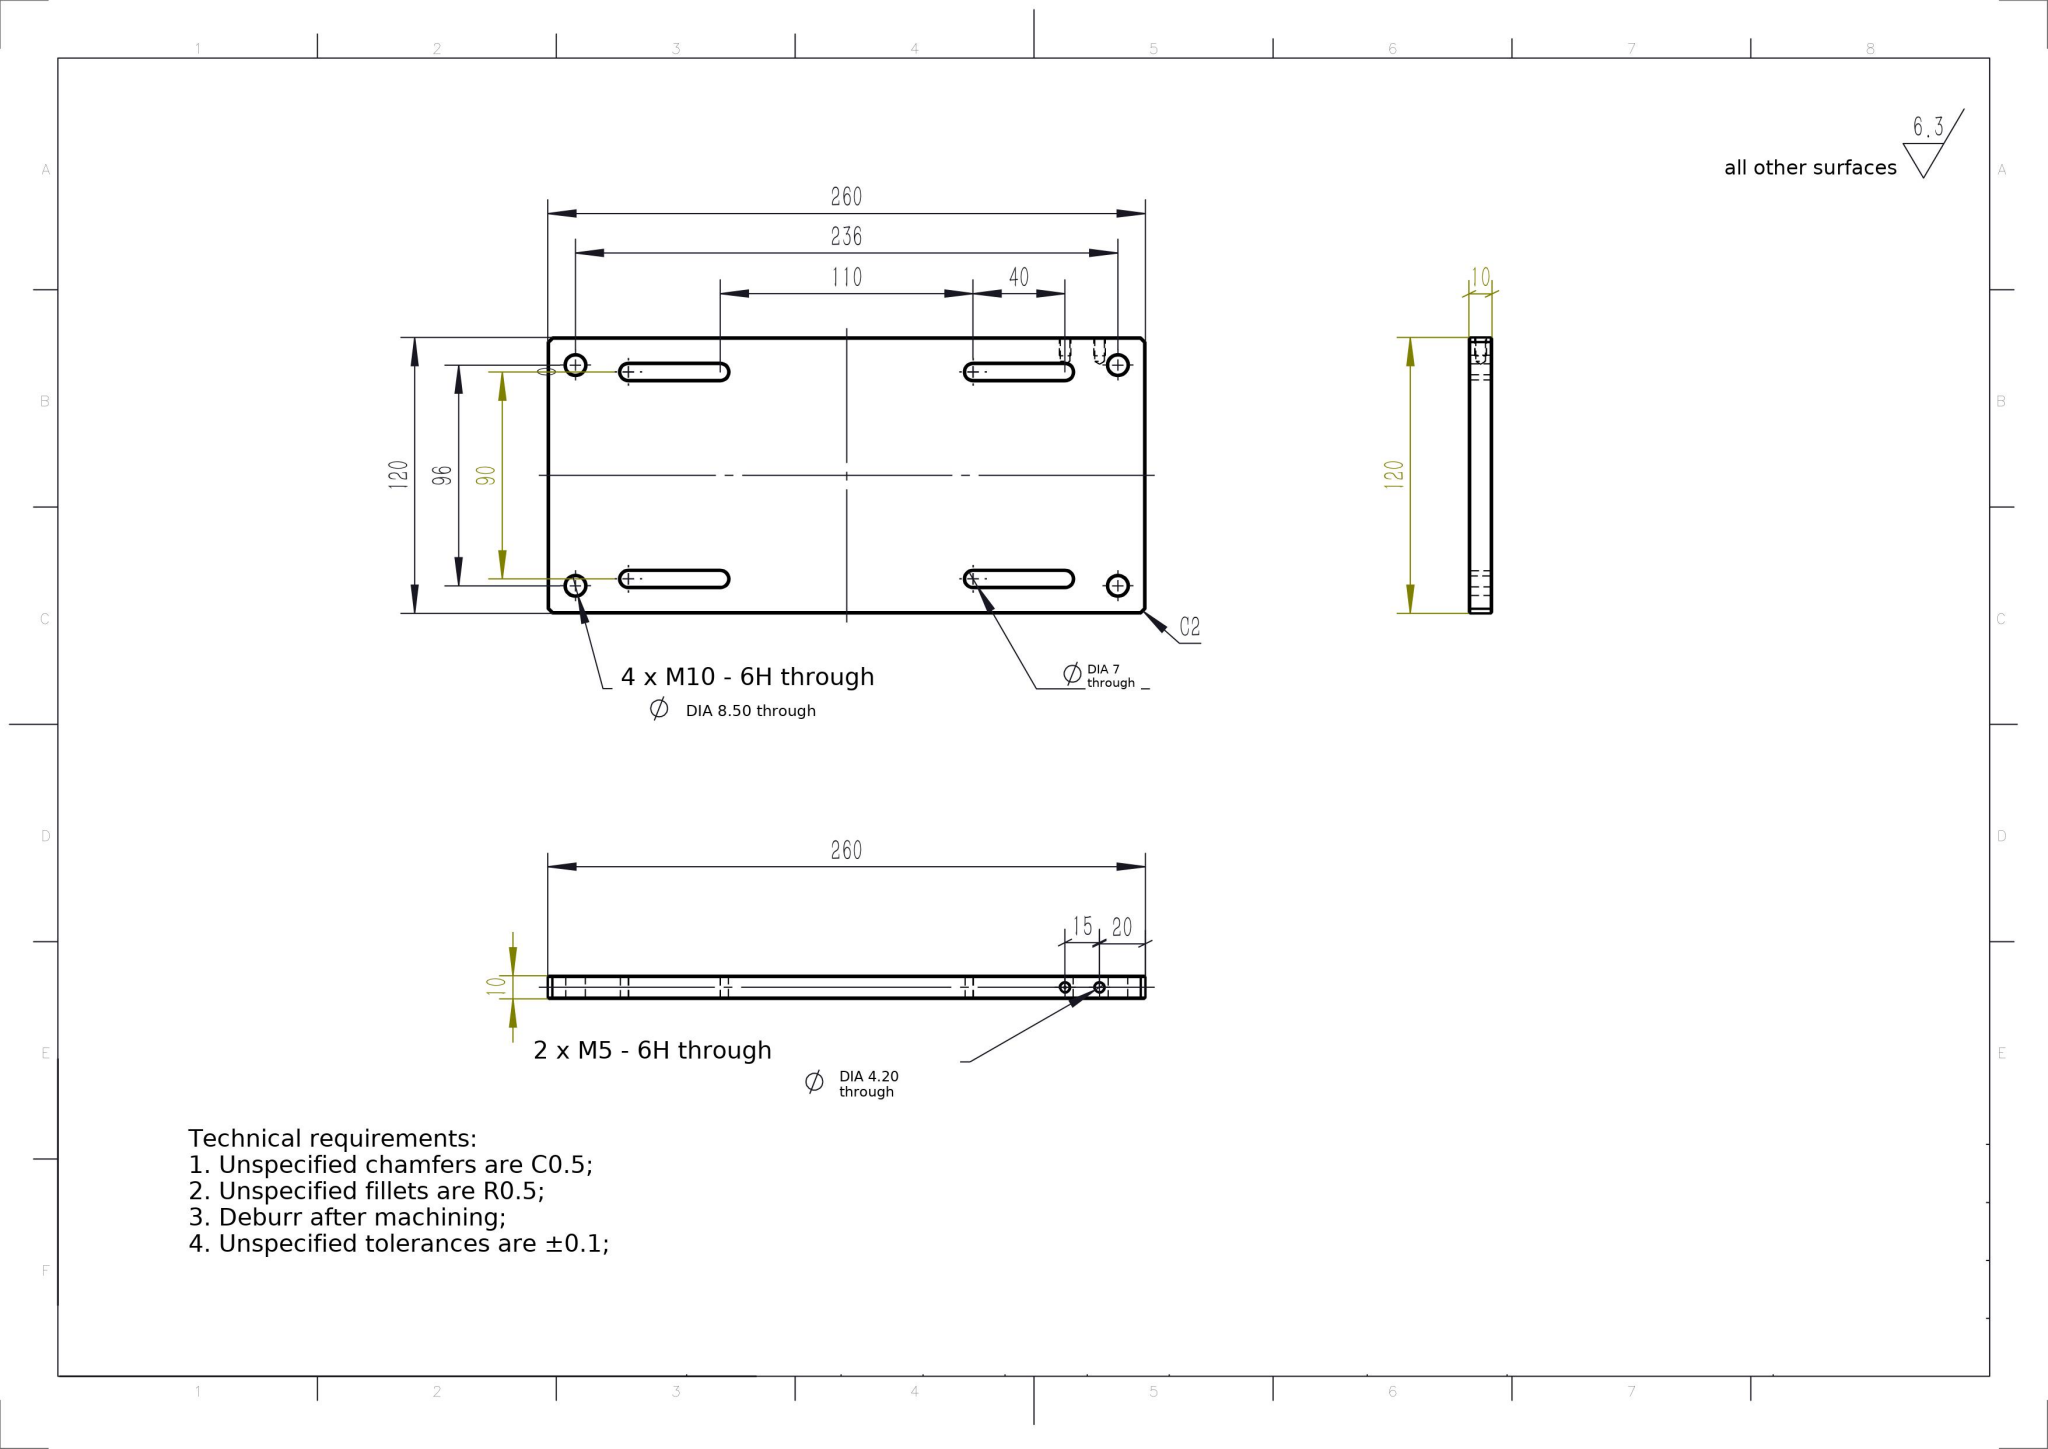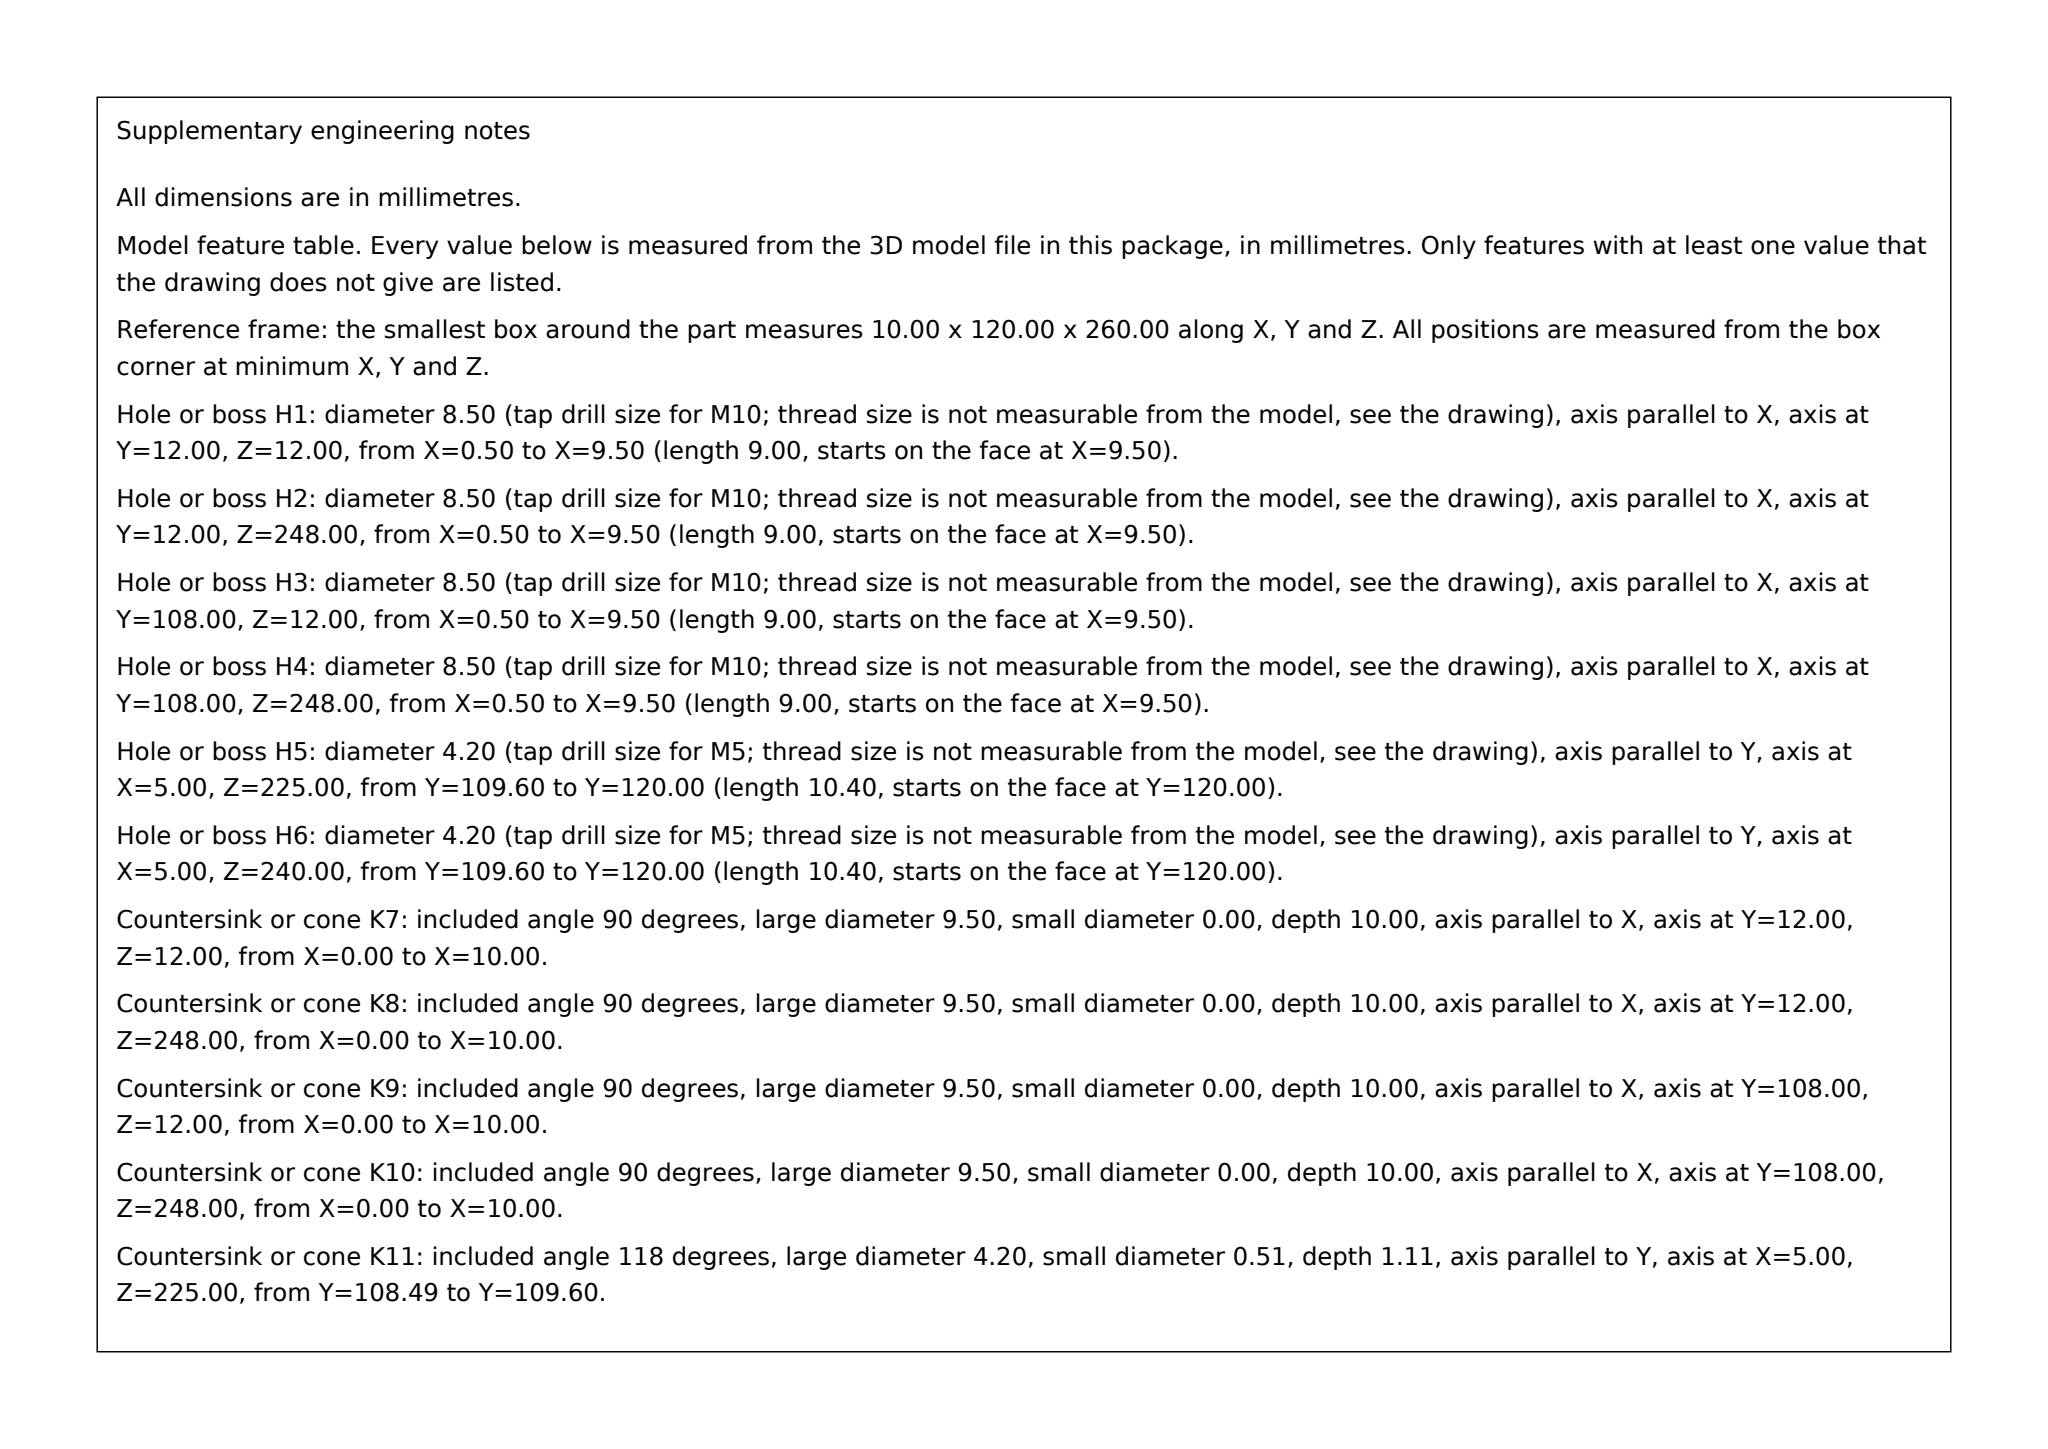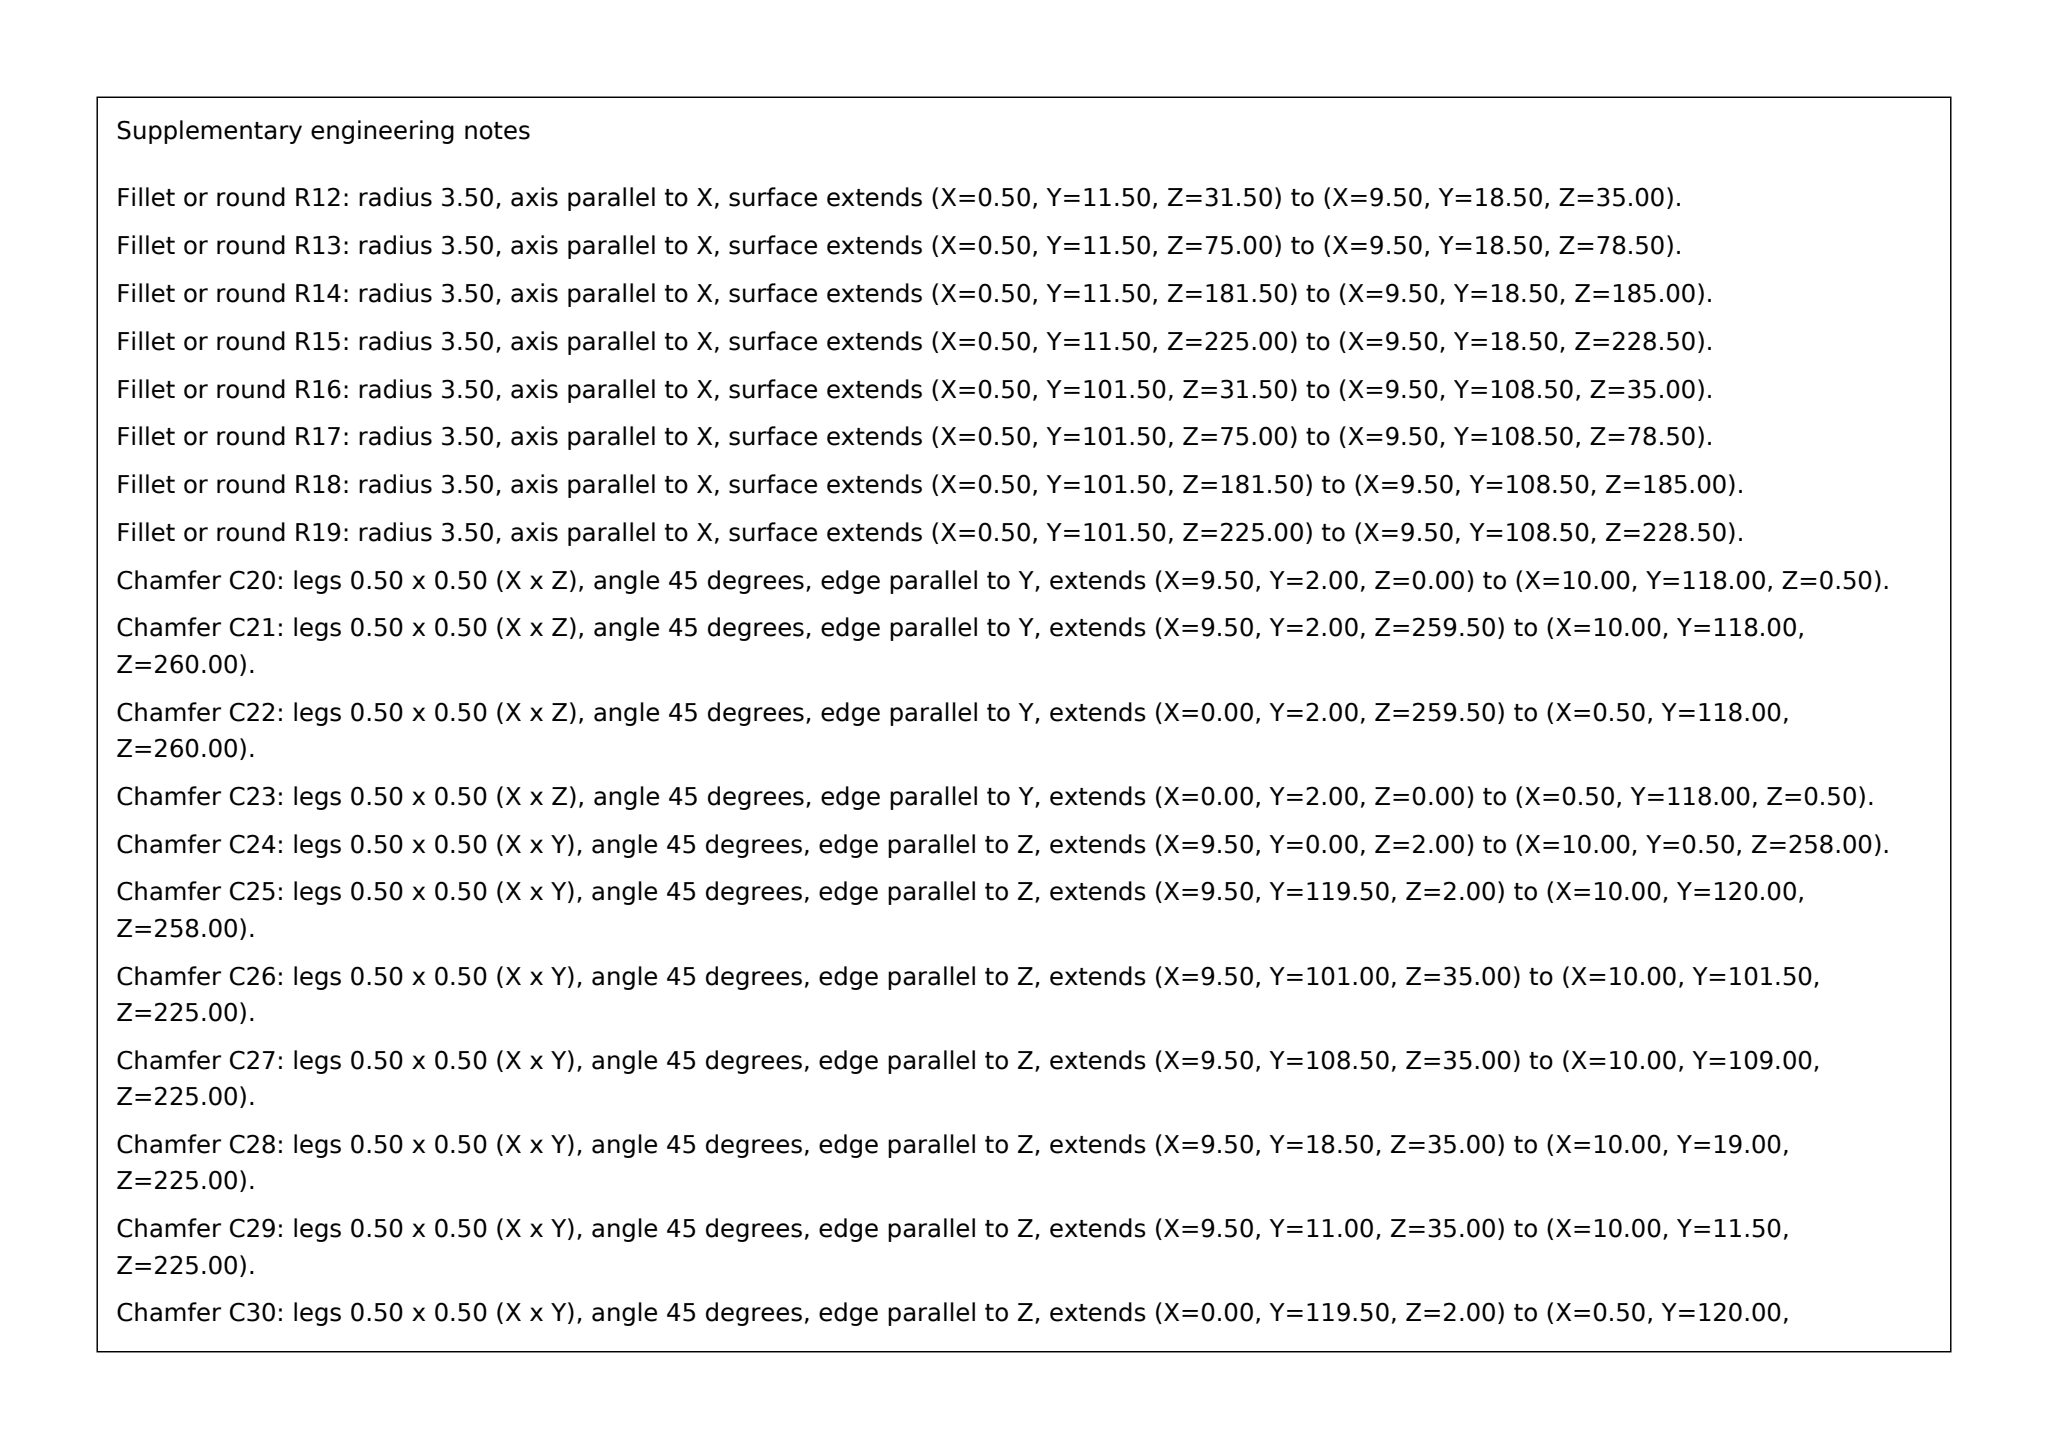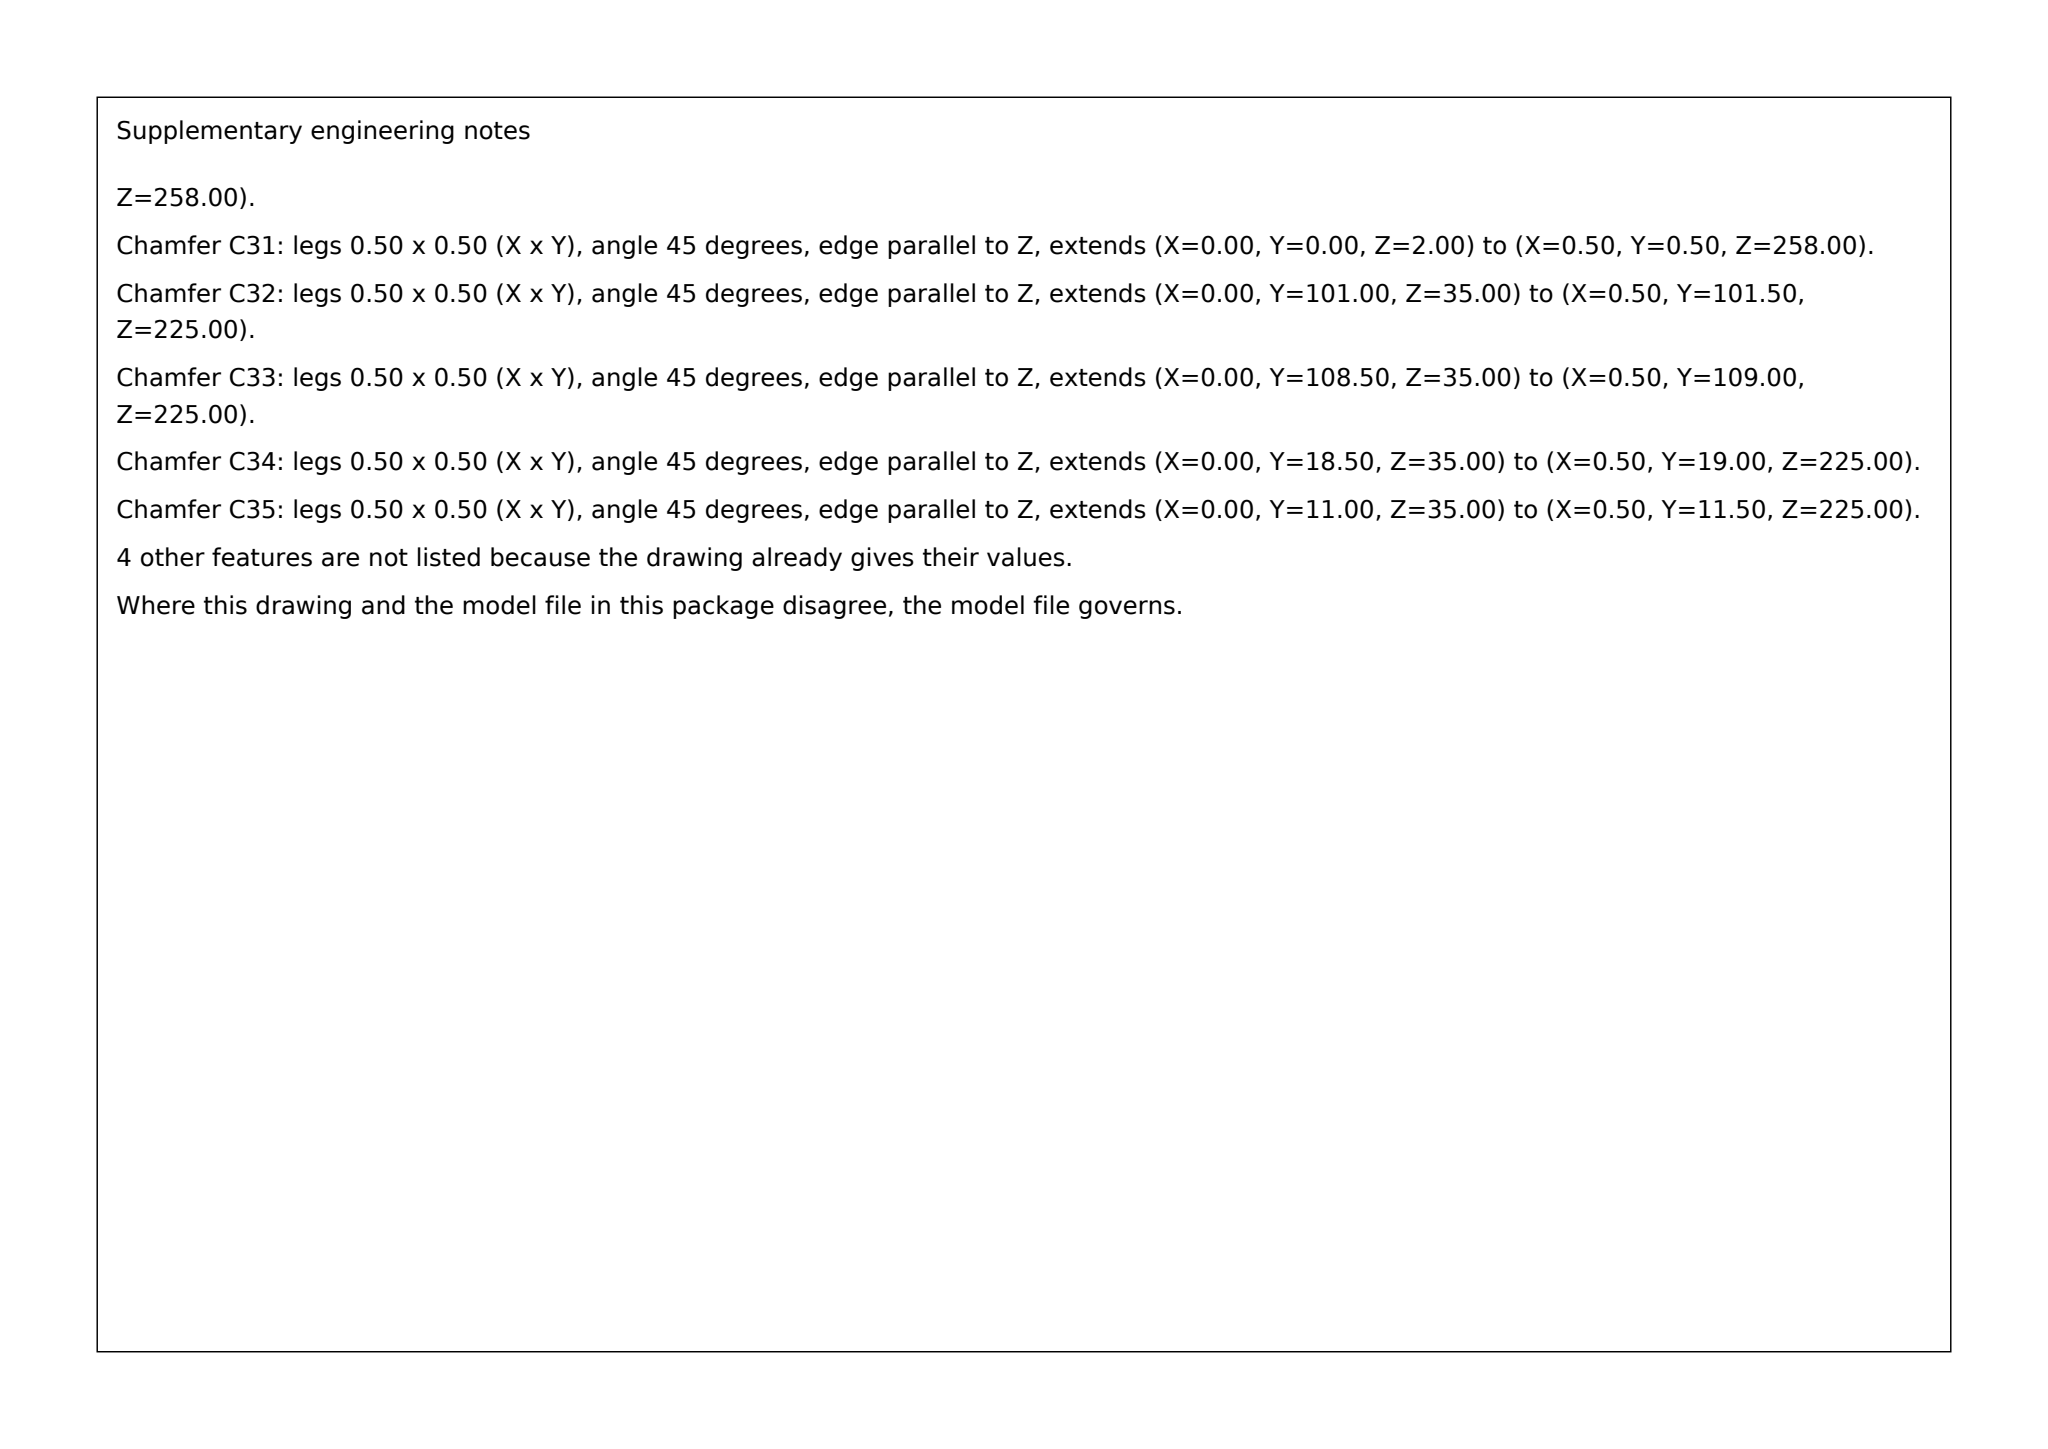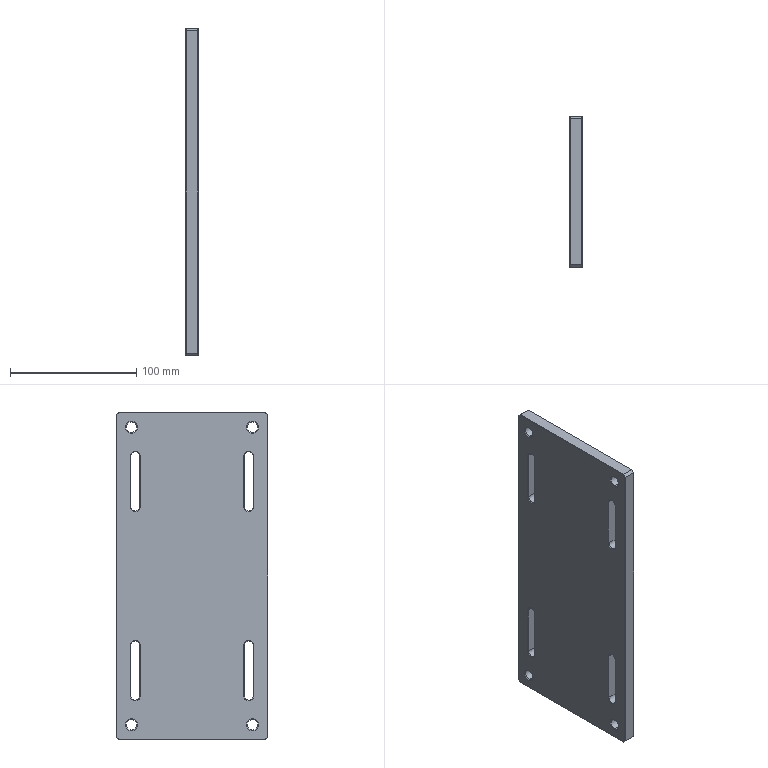Part | SolidWorks | mm | 1 solid | 118 faces | box 10 x 120 x 260 mm | volume 296292 mm3 | plane 50 | cone 44 | cylinder 24 | commonest cylinder face diameters 7 x12 8.5 x8 4.2 x4
build123d program:
from build123d import *

# Parameters (mm, degrees)
SKETCH2_W             = 260
SKETCH2_H             = 120
BOSS_EXTRUDE1_DEPTH   = 10
SKETCH3_R             = 2.5
CUT_EXTRUDE1_DEPTH    = 10
M10_TAPPED_HOLE1_D    = 8.5
CUT_EXTRUDE2_DEPTH    = 10
CHAMFER1_SIZE         = 2
M5_TAPPED_HOLE1_D     = 4.2
M5_TAPPED_HOLE1_DEPTH = 10.4
M5_TAPPED_HOLE1_TIP   = 1.262
CHAMFER2_SIZE         = 0.5


with BuildPart() as part:
    # Sketch2 → Boss-Extrude1 (new body)
    with BuildSketch(Plane(origin=(0, 0, 0), x_dir=(0, 0, -1), z_dir=(1, 0, 0))):
        Rectangle(SKETCH2_W, SKETCH2_H)
    extrude(amount=BOSS_EXTRUDE1_DEPTH)

    # Sketch3 → Cut-Extrude1 (cut)
    with BuildSketch(Plane(origin=(10, 0, 0), x_dir=(0, 0, -1), z_dir=(1, 0, 0))):
        with Locations((-118, 48)):
            Circle(SKETCH3_R)
        with Locations(Location((118, 48, 0), (0, 0, 180))):
            Circle(SKETCH3_R)
        with Locations((118, -48)):
            Circle(SKETCH3_R)
        with Locations(Location((-118, -48, 0), (0, 0, 180))):
            Circle(SKETCH3_R)
    extrude(amount=-CUT_EXTRUDE1_DEPTH, mode=Mode.SUBTRACT)

    # M10 Tapped Hole1 (through all)
    with Locations(Plane.ZY):
        with Locations((-118, 48), (-118, -48), (118, -48), (118, 48)):
            Hole(M10_TAPPED_HOLE1_D / 2)

    # Sketch6 → Cut-Extrude2 (cut)
    with BuildSketch(Plane.ZY):
        with BuildLine():
            Line((-95, 48.5), (-55, 48.5))
            ThreePointArc((-55, 48.5), (-51.5, 45), (-55, 41.5))
            Line((-55, 41.5), (-95, 41.5))
            ThreePointArc((-95, 41.5), (-98.5, 45), (-95, 48.5))
        make_face()
        with BuildLine():
            Line((-95, -48.5), (-55, -48.5))
            ThreePointArc((-55, -48.5), (-51.5, -45), (-55, -41.5))
            Line((-55, -41.5), (-95, -41.5))
            ThreePointArc((-95, -41.5), (-98.5, -45), (-95, -48.5))
        make_face()
        with BuildLine():
            Line((95, 48.5), (55, 48.5))
            ThreePointArc((55, 48.5), (51.5, 45), (55, 41.5))
            Line((55, 41.5), (95, 41.5))
            ThreePointArc((95, 41.5), (98.5, 45), (95, 48.5))
        make_face()
        with BuildLine():
            Line((95, -48.5), (55, -48.5))
            ThreePointArc((55, -48.5), (51.5, -45), (55, -41.5))
            Line((55, -41.5), (95, -41.5))
            ThreePointArc((95, -41.5), (98.5, -45), (95, -48.5))
        make_face()
    extrude(amount=-CUT_EXTRUDE2_DEPTH, mode=Mode.SUBTRACT)

    # Chamfer1
    chamfer1_edges = [part.edges().sort_by_distance(p)[0] for p in [
        (5, -60, -130),
        (5, -60, 130),
        (5, 60, 130),
        (5, 60, -130),
    ]]
    chamfer(chamfer1_edges, length=CHAMFER1_SIZE)

    # M5 Tapped Hole1
    with Locations(Plane(origin=(0, 60, 0), x_dir=(1, 0, 0), z_dir=(0, 1, 0))):
        with Locations((5, -95), (5, -110)):
            Hole(M5_TAPPED_HOLE1_D / 2, depth=M5_TAPPED_HOLE1_DEPTH)
            with Locations((0, 0, -(M5_TAPPED_HOLE1_DEPTH + M5_TAPPED_HOLE1_TIP / 2))):  # 118° drill point
                Cone(0, M5_TAPPED_HOLE1_D / 2, M5_TAPPED_HOLE1_TIP, mode=Mode.SUBTRACT)

    # Chamfer2
    chamfer2_edges = [part.edges().sort_by_distance(p)[0] for p in [
        (0, -60, 0),
        (10, -60, 0),
        (0, 0, -130),
        (0, 0, 130),
        (0, 60, 0),
        (0, -59, -129),
        (0, 59, -129),
        (0, 59, 129),
        (0, -59, 129),
        (10, 0, 130),
        (10, 0, -130),
        (10, 60, 0),
        (10, -59, -129),
        (10, 59, -129),
        (10, 59, 129),
        (10, -59, 129),
        (0, 48, 122.25),
        (10, 48, 122.25),
        (0, -48, 122.25),
        (10, -48, 122.25),
        (0, -48, -113.75),
        (10, -48, -113.75),
        (0, 48, -113.75),
        (10, 48, -113.75),
        (10, -45, -98.5),
        (10, -41.5, -75),
        (10, -45, -51.5),
        (10, -48.5, -75),
        (0, -45, -98.5),
        (0, -48.5, -75),
        (0, -45, -51.5),
        (0, -41.5, -75),
        (10, 45, 98.5),
        (10, 41.5, 75),
        (10, 45, 51.5),
        (10, 48.5, 75),
        (0, 45, 98.5),
        (0, 48.5, 75),
        (0, 45, 51.5),
        (0, 41.5, 75),
        (10, -45, 98.5),
        (10, -48.5, 75),
        (10, -45, 51.5),
        (10, -41.5, 75),
        (0, -45, 98.5),
        (0, -41.5, 75),
        (0, -45, 51.5),
        (0, -48.5, 75),
        (10, 45, -98.5),
        (10, 48.5, -75),
        (10, 45, -51.5),
        (10, 41.5, -75),
        (0, 45, -98.5),
        (0, 41.5, -75),
        (0, 45, -51.5),
        (0, 48.5, -75),
    ]]
    chamfer(chamfer2_edges, length=CHAMFER2_SIZE)


solid = part.part